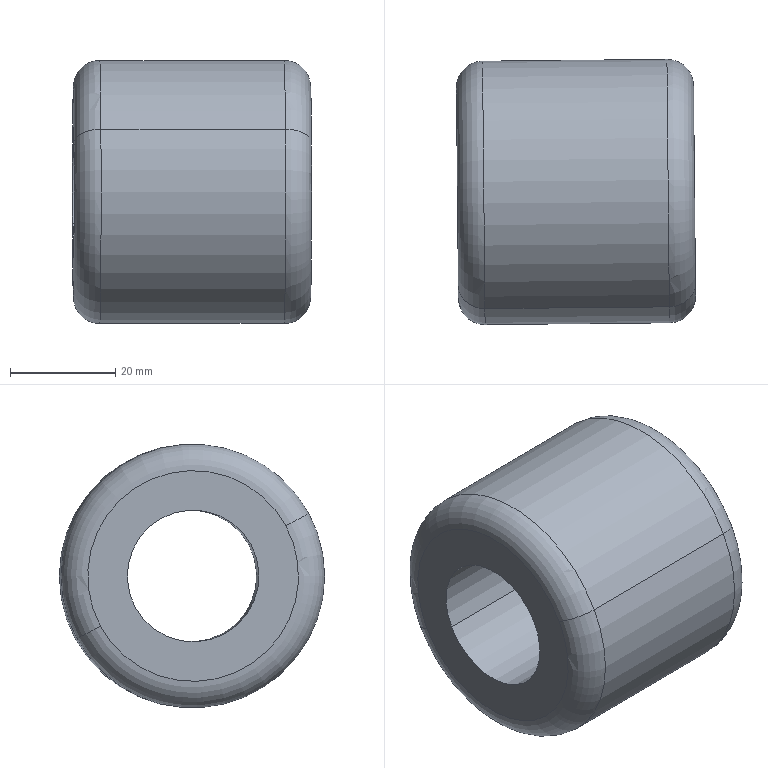Component | SolidWorks | CMAS50_F-2_CMAS50_Fwheel-1 | 1 solid | 10 faces | box 45.38 x 50.34 x 50 mm | volume 64658 mm3 | torus 4 | cylinder 4 | plane 2 | commonest cylinder face diameters 50 x2 25 x2 | material 45
build123d program:
from build123d import *


with BuildPart() as part:
    # Sketch1 → Revolve1 (revolve)
    with BuildSketch(Plane(origin=(0, 0, 0), x_dir=(0, 0, -1), z_dir=(1, 0, 0)), mode=Mode.PRIVATE) as revolve1_sk:
        with BuildLine():
            Line((-22.5, 12.5), (22.5, 12.5))
            Line((22.5, 12.5), (22.5, 20))
            ThreePointArc((22.5, 20), (21.036, 23.536), (17.5, 25))
            Line((17.5, 25), (-17.5, 25))
            ThreePointArc((-17.5, 25), (-21.036, 23.536), (-22.5, 20))
            Line((-22.5, 20), (-22.5, 12.5))
        make_face()
    revolve(revolve1_sk.sketch.rotate(Axis((0, 0, -22.5), (0, 0, 1)), 270), axis=Axis((0, 0, -22.5), (0, 0, 1)))


solid = part.part

# Placed as in the assembly
solid = solid.moved(Location((263.556, 604.998, 669), (-90, 89.448, -23.266)))
STEP:
#1=COLOUR_RGB('',0.7922,0.8196,0.9333);
#2=FILL_AREA_STYLE_COLOUR('',#1);
#3=FILL_AREA_STYLE('',(#2));
#4=SURFACE_STYLE_FILL_AREA(#3);
#5=SURFACE_SIDE_STYLE('',(#4));
#6=SURFACE_STYLE_USAGE(.BOTH.,#5);
#7=PRESENTATION_STYLE_ASSIGNMENT((#6));
#8=CARTESIAN_POINT('',(11.057,24.691,25.87));
#9=VERTEX_POINT('',#8);
#10=CARTESIAN_POINT('',(11.074,22.96,26.807));
#11=VERTEX_POINT('',#10);
#12=CARTESIAN_POINT('',(11.065,23.825,26.339));
#13=DIRECTION('',(1.,0.009642,0.));
#14=DIRECTION('',(-0.00848,0.8794,-0.476));
#15=AXIS2_PLACEMENT_3D('',#12,#13,#14);
#16=CIRCLE('',#15,0.9843);
#17=EDGE_CURVE('',#9,#11,#16,.T.);
#18=ORIENTED_EDGE('',*,*,#17,.T.);
#19=CARTESIAN_POINT('',(11.269,23.135,26.713));
#20=VERTEX_POINT('',#19);
#21=CARTESIAN_POINT('',(11.072,23.133,26.713));
#22=DIRECTION('',(-0.004589,0.4759,0.8795));
#23=DIRECTION('',(0.,-0.8795,0.476));
#24=AXIS2_PLACEMENT_3D('',#21,#22,#23);
#25=CIRCLE('',#24,0.1969);
#26=EDGE_CURVE('',#11,#20,#25,.T.);
#27=ORIENTED_EDGE('',*,*,#26,.T.);
#28=CARTESIAN_POINT('',(11.255,24.52,25.964));
#29=VERTEX_POINT('',#28);
#30=CARTESIAN_POINT('',(11.262,23.827,26.339));
#31=DIRECTION('',(1.,0.009642,0.));
#32=DIRECTION('',(-0.00848,0.8794,-0.476));
#33=AXIS2_PLACEMENT_3D('',#30,#31,#32);
#34=CIRCLE('',#33,0.7874);
#35=EDGE_CURVE('',#29,#20,#34,.T.);
#36=ORIENTED_EDGE('',*,*,#35,.F.);
#37=CARTESIAN_POINT('',(11.059,24.518,25.964));
#38=DIRECTION('',(0.004589,-0.4759,-0.8795));
#39=DIRECTION('',(0.,0.8795,-0.476));
#40=AXIS2_PLACEMENT_3D('',#37,#38,#39);
#41=CIRCLE('',#40,0.1969);
#42=EDGE_CURVE('',#9,#29,#41,.T.);
#43=ORIENTED_EDGE('',*,*,#42,.F.);
#44=EDGE_LOOP('',(#18,#27,#36,#43));
#45=FACE_OUTER_BOUND('',#44,.T.);
#46=CARTESIAN_POINT('',(11.065,23.825,26.339));
#47=DIRECTION('',(1.,0.009642,0.));
#48=DIRECTION('',(-0.00848,0.8794,-0.476));
#49=AXIS2_PLACEMENT_3D('',#46,#47,#48);
#50=TOROIDAL_SURFACE('',#49,0.7874,0.1969);
#51=ADVANCED_FACE('',(#45),#50,.T.);
#52=CARTESIAN_POINT('',(9.679,24.678,25.87));
#53=VERTEX_POINT('',#52);
#54=CARTESIAN_POINT('',(9.696,22.947,26.807));
#55=VERTEX_POINT('',#54);
#56=CARTESIAN_POINT('',(9.687,23.812,26.339));
#57=DIRECTION('',(1.,0.009642,0.));
#58=DIRECTION('',(-0.00848,0.8794,-0.476));
#59=AXIS2_PLACEMENT_3D('',#56,#57,#58);
#60=CIRCLE('',#59,0.9843);
#61=EDGE_CURVE('',#53,#55,#60,.T.);
#62=ORIENTED_EDGE('',*,*,#61,.T.);
#63=CARTESIAN_POINT('',(9.499,22.945,26.807));
#64=DIRECTION('',(1.,0.009642,0.));
#65=VECTOR('',#64,39.37);
#66=LINE('',#63,#65);
#67=EDGE_CURVE('',#55,#11,#66,.T.);
#68=ORIENTED_EDGE('',*,*,#67,.T.);
#69=ORIENTED_EDGE('',*,*,#17,.F.);
#70=CARTESIAN_POINT('',(9.482,24.676,25.87));
#71=DIRECTION('',(1.,0.009642,0.));
#72=VECTOR('',#71,39.37);
#73=LINE('',#70,#72);
#74=EDGE_CURVE('',#53,#9,#73,.T.);
#75=ORIENTED_EDGE('',*,*,#74,.F.);
#76=EDGE_LOOP('',(#62,#68,#69,#75));
#77=FACE_OUTER_BOUND('',#76,.T.);
#78=CARTESIAN_POINT('',(9.49,23.81,26.339));
#79=DIRECTION('',(1.,0.009642,0.));
#80=DIRECTION('',(-0.00848,0.8794,-0.476));
#81=AXIS2_PLACEMENT_3D('',#78,#79,#80);
#82=CYLINDRICAL_SURFACE('',#81,0.9843);
#83=ADVANCED_FACE('',(#77),#82,.T.);
#84=CARTESIAN_POINT('',(9.484,24.503,25.964));
#85=VERTEX_POINT('',#84);
#86=CARTESIAN_POINT('',(9.497,23.118,26.713));
#87=VERTEX_POINT('',#86);
#88=CARTESIAN_POINT('',(9.49,23.81,26.339));
#89=DIRECTION('',(1.,0.009642,0.));
#90=DIRECTION('',(-0.00848,0.8794,-0.476));
#91=AXIS2_PLACEMENT_3D('',#88,#89,#90);
#92=CIRCLE('',#91,0.7874);
#93=EDGE_CURVE('',#85,#87,#92,.T.);
#94=ORIENTED_EDGE('',*,*,#93,.T.);
#95=CARTESIAN_POINT('',(9.694,23.12,26.713));
#96=DIRECTION('',(-0.004589,0.4759,0.8795));
#97=DIRECTION('',(0.,-0.8795,0.476));
#98=AXIS2_PLACEMENT_3D('',#95,#96,#97);
#99=CIRCLE('',#98,0.1969);
#100=EDGE_CURVE('',#87,#55,#99,.T.);
#101=ORIENTED_EDGE('',*,*,#100,.T.);
#102=ORIENTED_EDGE('',*,*,#61,.F.);
#103=CARTESIAN_POINT('',(9.681,24.505,25.964));
#104=DIRECTION('',(0.004589,-0.4759,-0.8795));
#105=DIRECTION('',(0.,0.8795,-0.476));
#106=AXIS2_PLACEMENT_3D('',#103,#104,#105);
#107=CIRCLE('',#106,0.1969);
#108=EDGE_CURVE('',#85,#53,#107,.T.);
#109=ORIENTED_EDGE('',*,*,#108,.F.);
#110=EDGE_LOOP('',(#94,#101,#102,#109));
#111=FACE_OUTER_BOUND('',#110,.T.);
#112=CARTESIAN_POINT('',(9.687,23.812,26.339));
#113=DIRECTION('',(1.,0.009642,0.));
#114=DIRECTION('',(-0.00848,0.8794,-0.476));
#115=AXIS2_PLACEMENT_3D('',#112,#113,#114);
#116=TOROIDAL_SURFACE('',#115,0.7874,0.1969);
#117=ADVANCED_FACE('',(#111),#116,.T.);
#118=CARTESIAN_POINT('',(9.495,23.377,26.573));
#119=VERTEX_POINT('',#118);
#120=CARTESIAN_POINT('',(9.486,24.243,26.104));
#121=VERTEX_POINT('',#120);
#122=CARTESIAN_POINT('',(9.49,23.81,26.339));
#123=DIRECTION('',(1.,0.009642,0.));
#124=DIRECTION('',(-0.00848,0.8794,-0.476));
#125=AXIS2_PLACEMENT_3D('',#122,#123,#124);
#126=CIRCLE('',#125,0.4921);
#127=EDGE_CURVE('',#119,#121,#126,.T.);
#128=ORIENTED_EDGE('',*,*,#127,.F.);
#129=CARTESIAN_POINT('',(11.266,23.395,26.573));
#130=VERTEX_POINT('',#129);
#131=CARTESIAN_POINT('',(9.495,23.377,26.573));
#132=DIRECTION('',(1.,0.009642,0.));
#133=VECTOR('',#132,39.37);
#134=LINE('',#131,#133);
#135=EDGE_CURVE('',#119,#130,#134,.T.);
#136=ORIENTED_EDGE('',*,*,#135,.T.);
#137=CARTESIAN_POINT('',(11.258,24.26,26.104));
#138=VERTEX_POINT('',#137);
#139=CARTESIAN_POINT('',(11.262,23.827,26.339));
#140=DIRECTION('',(1.,0.009642,0.));
#141=DIRECTION('',(-0.00848,0.8794,-0.476));
#142=AXIS2_PLACEMENT_3D('',#139,#140,#141);
#143=CIRCLE('',#142,0.4921);
#144=EDGE_CURVE('',#130,#138,#143,.T.);
#145=ORIENTED_EDGE('',*,*,#144,.T.);
#146=CARTESIAN_POINT('',(9.486,24.243,26.104));
#147=DIRECTION('',(1.,0.009642,0.));
#148=VECTOR('',#147,39.37);
#149=LINE('',#146,#148);
#150=EDGE_CURVE('',#121,#138,#149,.T.);
#151=ORIENTED_EDGE('',*,*,#150,.F.);
#152=EDGE_LOOP('',(#128,#136,#145,#151));
#153=FACE_OUTER_BOUND('',#152,.T.);
#154=CARTESIAN_POINT('',(9.49,23.81,26.339));
#155=DIRECTION('',(1.,0.009642,0.));
#156=DIRECTION('',(-0.00848,0.8794,-0.476));
#157=AXIS2_PLACEMENT_3D('',#154,#155,#156);
#158=CYLINDRICAL_SURFACE('',#157,0.4921);
#159=ADVANCED_FACE('',(#153),#158,.F.);
#160=CARTESIAN_POINT('',(11.262,23.827,26.339));
#161=DIRECTION('',(1.,0.009642,0.));
#162=DIRECTION('',(-0.00848,0.8794,-0.476));
#163=AXIS2_PLACEMENT_3D('',#160,#161,#162);
#164=CIRCLE('',#163,0.4921);
#165=EDGE_CURVE('',#138,#130,#164,.T.);
#166=ORIENTED_EDGE('',*,*,#165,.F.);
#167=ORIENTED_EDGE('',*,*,#144,.F.);
#168=EDGE_LOOP('',(#166,#167));
#169=FACE_BOUND('',#168,.T.);
#170=ORIENTED_EDGE('',*,*,#35,.T.);
#171=CARTESIAN_POINT('',(11.262,23.827,26.339));
#172=DIRECTION('',(1.,0.009642,0.));
#173=DIRECTION('',(-0.00848,0.8794,-0.476));
#174=AXIS2_PLACEMENT_3D('',#171,#172,#173);
#175=CIRCLE('',#174,0.7874);
#176=EDGE_CURVE('',#20,#29,#175,.T.);
#177=ORIENTED_EDGE('',*,*,#176,.T.);
#178=EDGE_LOOP('',(#170,#177));
#179=FACE_OUTER_BOUND('',#178,.T.);
#180=CARTESIAN_POINT('',(11.258,24.202,27.031));
#181=DIRECTION('',(-1.,-0.009642,-0.));
#182=DIRECTION('',(0.00848,-0.8794,0.476));
#183=AXIS2_PLACEMENT_3D('',#180,#181,#182);
#184=PLANE('',#183);
#185=ADVANCED_FACE('',(#169,#179),#184,.F.);
#186=ORIENTED_EDGE('',*,*,#135,.F.);
#187=CARTESIAN_POINT('',(9.49,23.81,26.339));
#188=DIRECTION('',(1.,0.009642,0.));
#189=DIRECTION('',(-0.00848,0.8794,-0.476));
#190=AXIS2_PLACEMENT_3D('',#187,#188,#189);
#191=CIRCLE('',#190,0.4921);
#192=EDGE_CURVE('',#121,#119,#191,.T.);
#193=ORIENTED_EDGE('',*,*,#192,.F.);
#194=ORIENTED_EDGE('',*,*,#150,.T.);
#195=ORIENTED_EDGE('',*,*,#165,.T.);
#196=EDGE_LOOP('',(#186,#193,#194,#195));
#197=FACE_OUTER_BOUND('',#196,.T.);
#198=CARTESIAN_POINT('',(9.49,23.81,26.339));
#199=DIRECTION('',(1.,0.009642,0.));
#200=DIRECTION('',(-0.00848,0.8794,-0.476));
#201=AXIS2_PLACEMENT_3D('',#198,#199,#200);
#202=CYLINDRICAL_SURFACE('',#201,0.4921);
#203=ADVANCED_FACE('',(#197),#202,.F.);
#204=ORIENTED_EDGE('',*,*,#93,.F.);
#205=CARTESIAN_POINT('',(9.49,23.81,26.339));
#206=DIRECTION('',(1.,0.009642,0.));
#207=DIRECTION('',(-0.00848,0.8794,-0.476));
#208=AXIS2_PLACEMENT_3D('',#205,#206,#207);
#209=CIRCLE('',#208,0.7874);
#210=EDGE_CURVE('',#87,#85,#209,.T.);
#211=ORIENTED_EDGE('',*,*,#210,.F.);
#212=EDGE_LOOP('',(#204,#211));
#213=FACE_OUTER_BOUND('',#212,.T.);
#214=ORIENTED_EDGE('',*,*,#192,.T.);
#215=ORIENTED_EDGE('',*,*,#127,.T.);
#216=EDGE_LOOP('',(#214,#215));
#217=FACE_BOUND('',#216,.T.);
#218=CARTESIAN_POINT('',(9.488,24.044,26.771));
#219=DIRECTION('',(1.,0.009642,0.));
#220=DIRECTION('',(-0.00848,0.8794,-0.476));
#221=AXIS2_PLACEMENT_3D('',#218,#219,#220);
#222=PLANE('',#221);
#223=ADVANCED_FACE('',(#213,#217),#222,.F.);
#224=ORIENTED_EDGE('',*,*,#100,.F.);
#225=ORIENTED_EDGE('',*,*,#210,.T.);
#226=ORIENTED_EDGE('',*,*,#108,.T.);
#227=CARTESIAN_POINT('',(9.687,23.812,26.339));
#228=DIRECTION('',(1.,0.009642,0.));
#229=DIRECTION('',(-0.00848,0.8794,-0.476));
#230=AXIS2_PLACEMENT_3D('',#227,#228,#229);
#231=CIRCLE('',#230,0.9843);
#232=EDGE_CURVE('',#55,#53,#231,.T.);
#233=ORIENTED_EDGE('',*,*,#232,.F.);
#234=EDGE_LOOP('',(#224,#225,#226,#233));
#235=FACE_OUTER_BOUND('',#234,.T.);
#236=CARTESIAN_POINT('',(9.687,23.812,26.339));
#237=DIRECTION('',(1.,0.009642,0.));
#238=DIRECTION('',(-0.00848,0.8794,-0.476));
#239=AXIS2_PLACEMENT_3D('',#236,#237,#238);
#240=TOROIDAL_SURFACE('',#239,0.7874,0.1969);
#241=ADVANCED_FACE('',(#235),#240,.T.);
#242=ORIENTED_EDGE('',*,*,#67,.F.);
#243=ORIENTED_EDGE('',*,*,#232,.T.);
#244=ORIENTED_EDGE('',*,*,#74,.T.);
#245=CARTESIAN_POINT('',(11.065,23.825,26.339));
#246=DIRECTION('',(1.,0.009642,0.));
#247=DIRECTION('',(-0.00848,0.8794,-0.476));
#248=AXIS2_PLACEMENT_3D('',#245,#246,#247);
#249=CIRCLE('',#248,0.9843);
#250=EDGE_CURVE('',#11,#9,#249,.T.);
#251=ORIENTED_EDGE('',*,*,#250,.F.);
#252=EDGE_LOOP('',(#242,#243,#244,#251));
#253=FACE_OUTER_BOUND('',#252,.T.);
#254=CARTESIAN_POINT('',(9.49,23.81,26.339));
#255=DIRECTION('',(1.,0.009642,0.));
#256=DIRECTION('',(-0.00848,0.8794,-0.476));
#257=AXIS2_PLACEMENT_3D('',#254,#255,#256);
#258=CYLINDRICAL_SURFACE('',#257,0.9843);
#259=ADVANCED_FACE('',(#253),#258,.T.);
#260=ORIENTED_EDGE('',*,*,#26,.F.);
#261=ORIENTED_EDGE('',*,*,#250,.T.);
#262=ORIENTED_EDGE('',*,*,#42,.T.);
#263=ORIENTED_EDGE('',*,*,#176,.F.);
#264=EDGE_LOOP('',(#260,#261,#262,#263));
#265=FACE_OUTER_BOUND('',#264,.T.);
#266=CARTESIAN_POINT('',(11.065,23.825,26.339));
#267=DIRECTION('',(1.,0.009642,0.));
#268=DIRECTION('',(-0.00848,0.8794,-0.476));
#269=AXIS2_PLACEMENT_3D('',#266,#267,#268);
#270=TOROIDAL_SURFACE('',#269,0.7874,0.1969);
#271=ADVANCED_FACE('',(#265),#270,.T.);
#272=CLOSED_SHELL('',(#51,#83,#117,#159,#185,#203,#223,#241,#259,#271));
#273=MANIFOLD_SOLID_BREP('',#272);
#274=STYLED_ITEM('',(#7),#273);
#275=PRESENTATION_LAYER_ASSIGNMENT('','',(#274));
#276=CARTESIAN_POINT('',(0.,0.,0.));
#277=DIRECTION('',(0.,0.,1.));
#278=DIRECTION('',(1.,0.,0.));
#279=AXIS2_PLACEMENT_3D('',#276,#277,#278);
#280=(LENGTH_UNIT()NAMED_UNIT(*)SI_UNIT($,.METRE.));
#281=LENGTH_MEASURE_WITH_UNIT(LENGTH_MEASURE(0.0254),#280);
#282=DIMENSIONAL_EXPONENTS(1.,0.,0.,0.,0.,0.,0.);
#283=(CONVERSION_BASED_UNIT('',#281)LENGTH_UNIT()NAMED_UNIT(#282));
#284=UNCERTAINTY_MEASURE_WITH_UNIT(LENGTH_MEASURE(0.00001),#283,'','');
#285=(NAMED_UNIT(*)PLANE_ANGLE_UNIT()SI_UNIT($,.RADIAN.));
#286=(NAMED_UNIT(*)SI_UNIT($,.STERADIAN.)SOLID_ANGLE_UNIT());
#287=(GEOMETRIC_REPRESENTATION_CONTEXT(3)GLOBAL_UNCERTAINTY_ASSIGNED_CONTEXT((#284))GLOBAL_UNIT_ASSIGNED_CONTEXT((#283,#285,#286))REPRESENTATION_CONTEXT('',''));
#288=ADVANCED_BREP_SHAPE_REPRESENTATION('',(#273,#279),#287);
#289=(LENGTH_UNIT()NAMED_UNIT(*)SI_UNIT($,.METRE.));
#290=LENGTH_MEASURE_WITH_UNIT(LENGTH_MEASURE(0.0254),#289);
#291=DIMENSIONAL_EXPONENTS(1.,0.,0.,0.,0.,0.,0.);
#292=(CONVERSION_BASED_UNIT('',#290)LENGTH_UNIT()NAMED_UNIT(#291));
#293=UNCERTAINTY_MEASURE_WITH_UNIT(LENGTH_MEASURE(0.00001),#292,'','');
#294=(NAMED_UNIT(*)PLANE_ANGLE_UNIT()SI_UNIT($,.RADIAN.));
#295=(NAMED_UNIT(*)SI_UNIT($,.STERADIAN.)SOLID_ANGLE_UNIT());
#296=(GEOMETRIC_REPRESENTATION_CONTEXT(3)GLOBAL_UNCERTAINTY_ASSIGNED_CONTEXT((#293))GLOBAL_UNIT_ASSIGNED_CONTEXT((#292,#294,#295))REPRESENTATION_CONTEXT('',''));
#297=MECHANICAL_DESIGN_GEOMETRIC_PRESENTATION_REPRESENTATION('',(#274),#296);